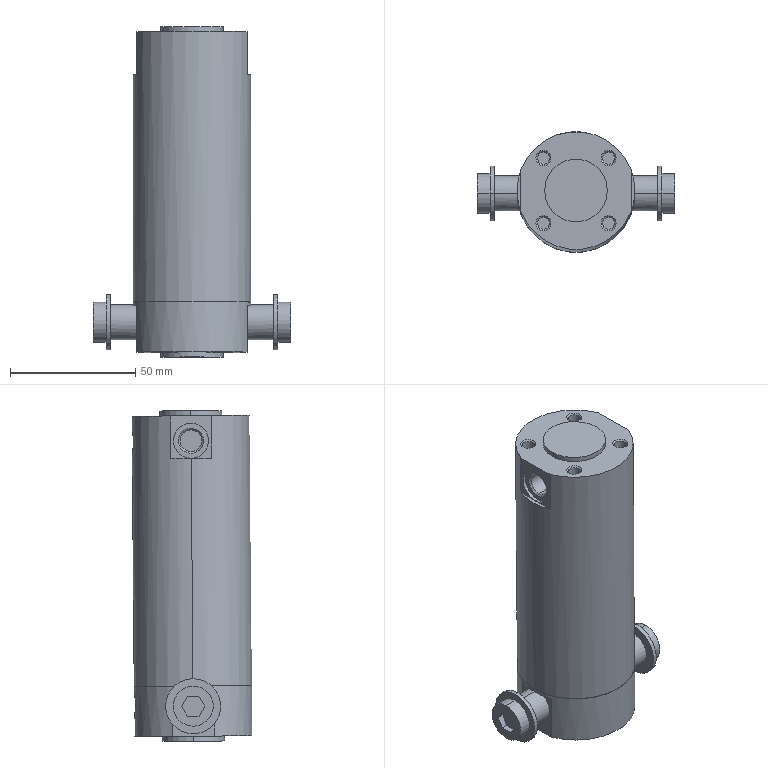Component | SolidWorks | CG1UN40-50CylinderBlock-1 | 1 solid | 130 faces | volume 151623 mm3 | cylinder 54 | plane 52 | cone 24 | commonest cylinder face diameters 4.917 x16 14 x8 16 x6 47 x4 25 x4 8.566 x4 8.647 x4 22 x4